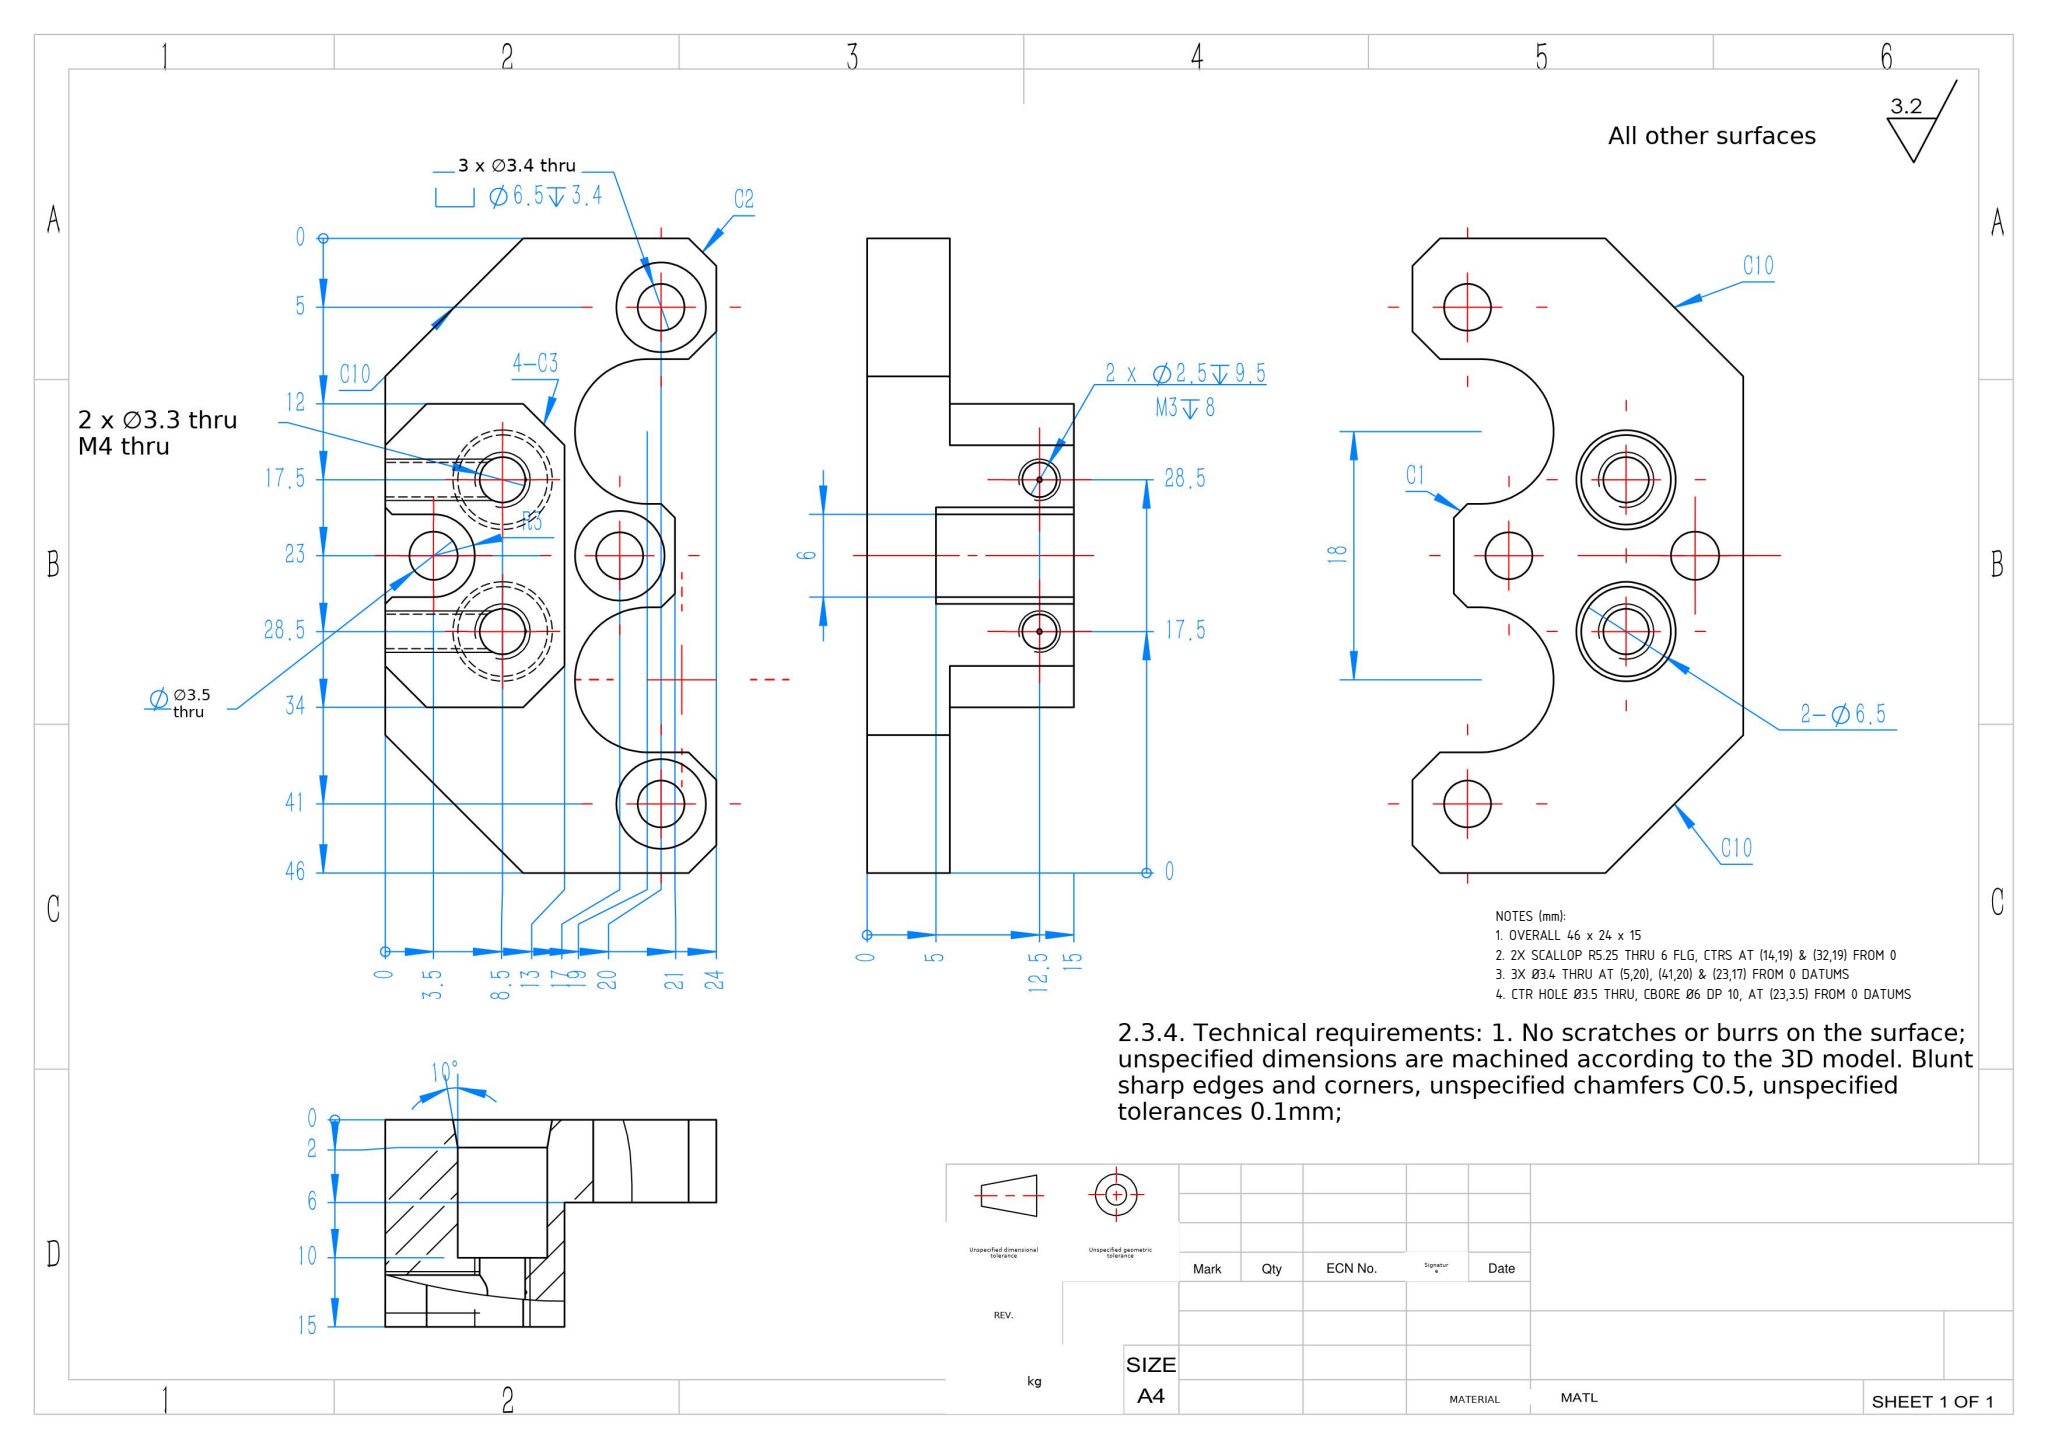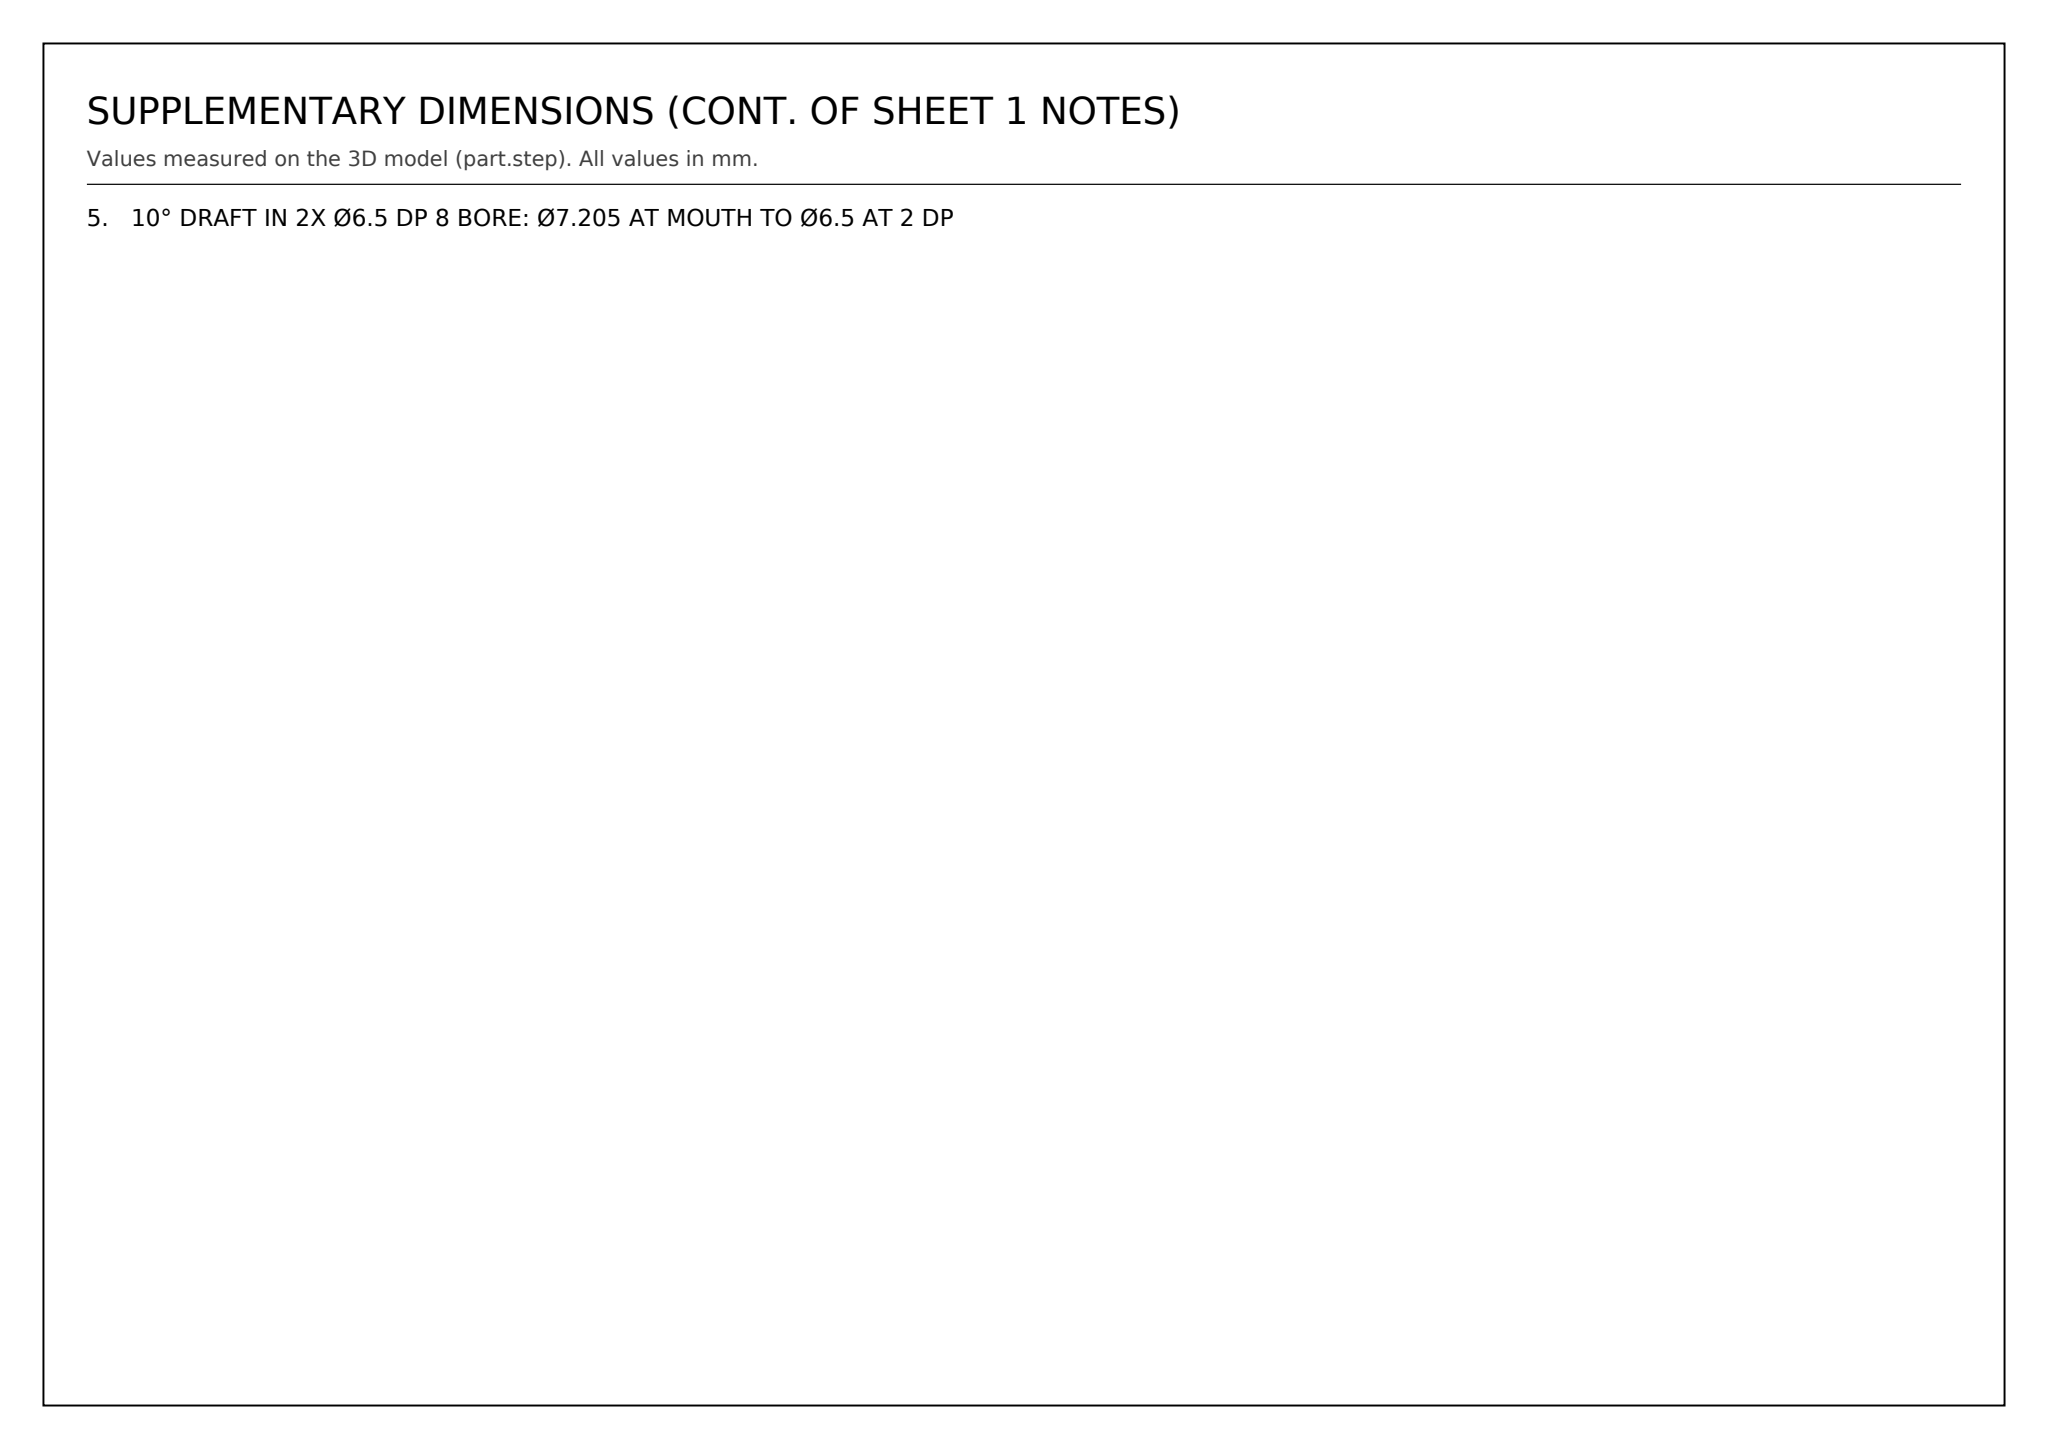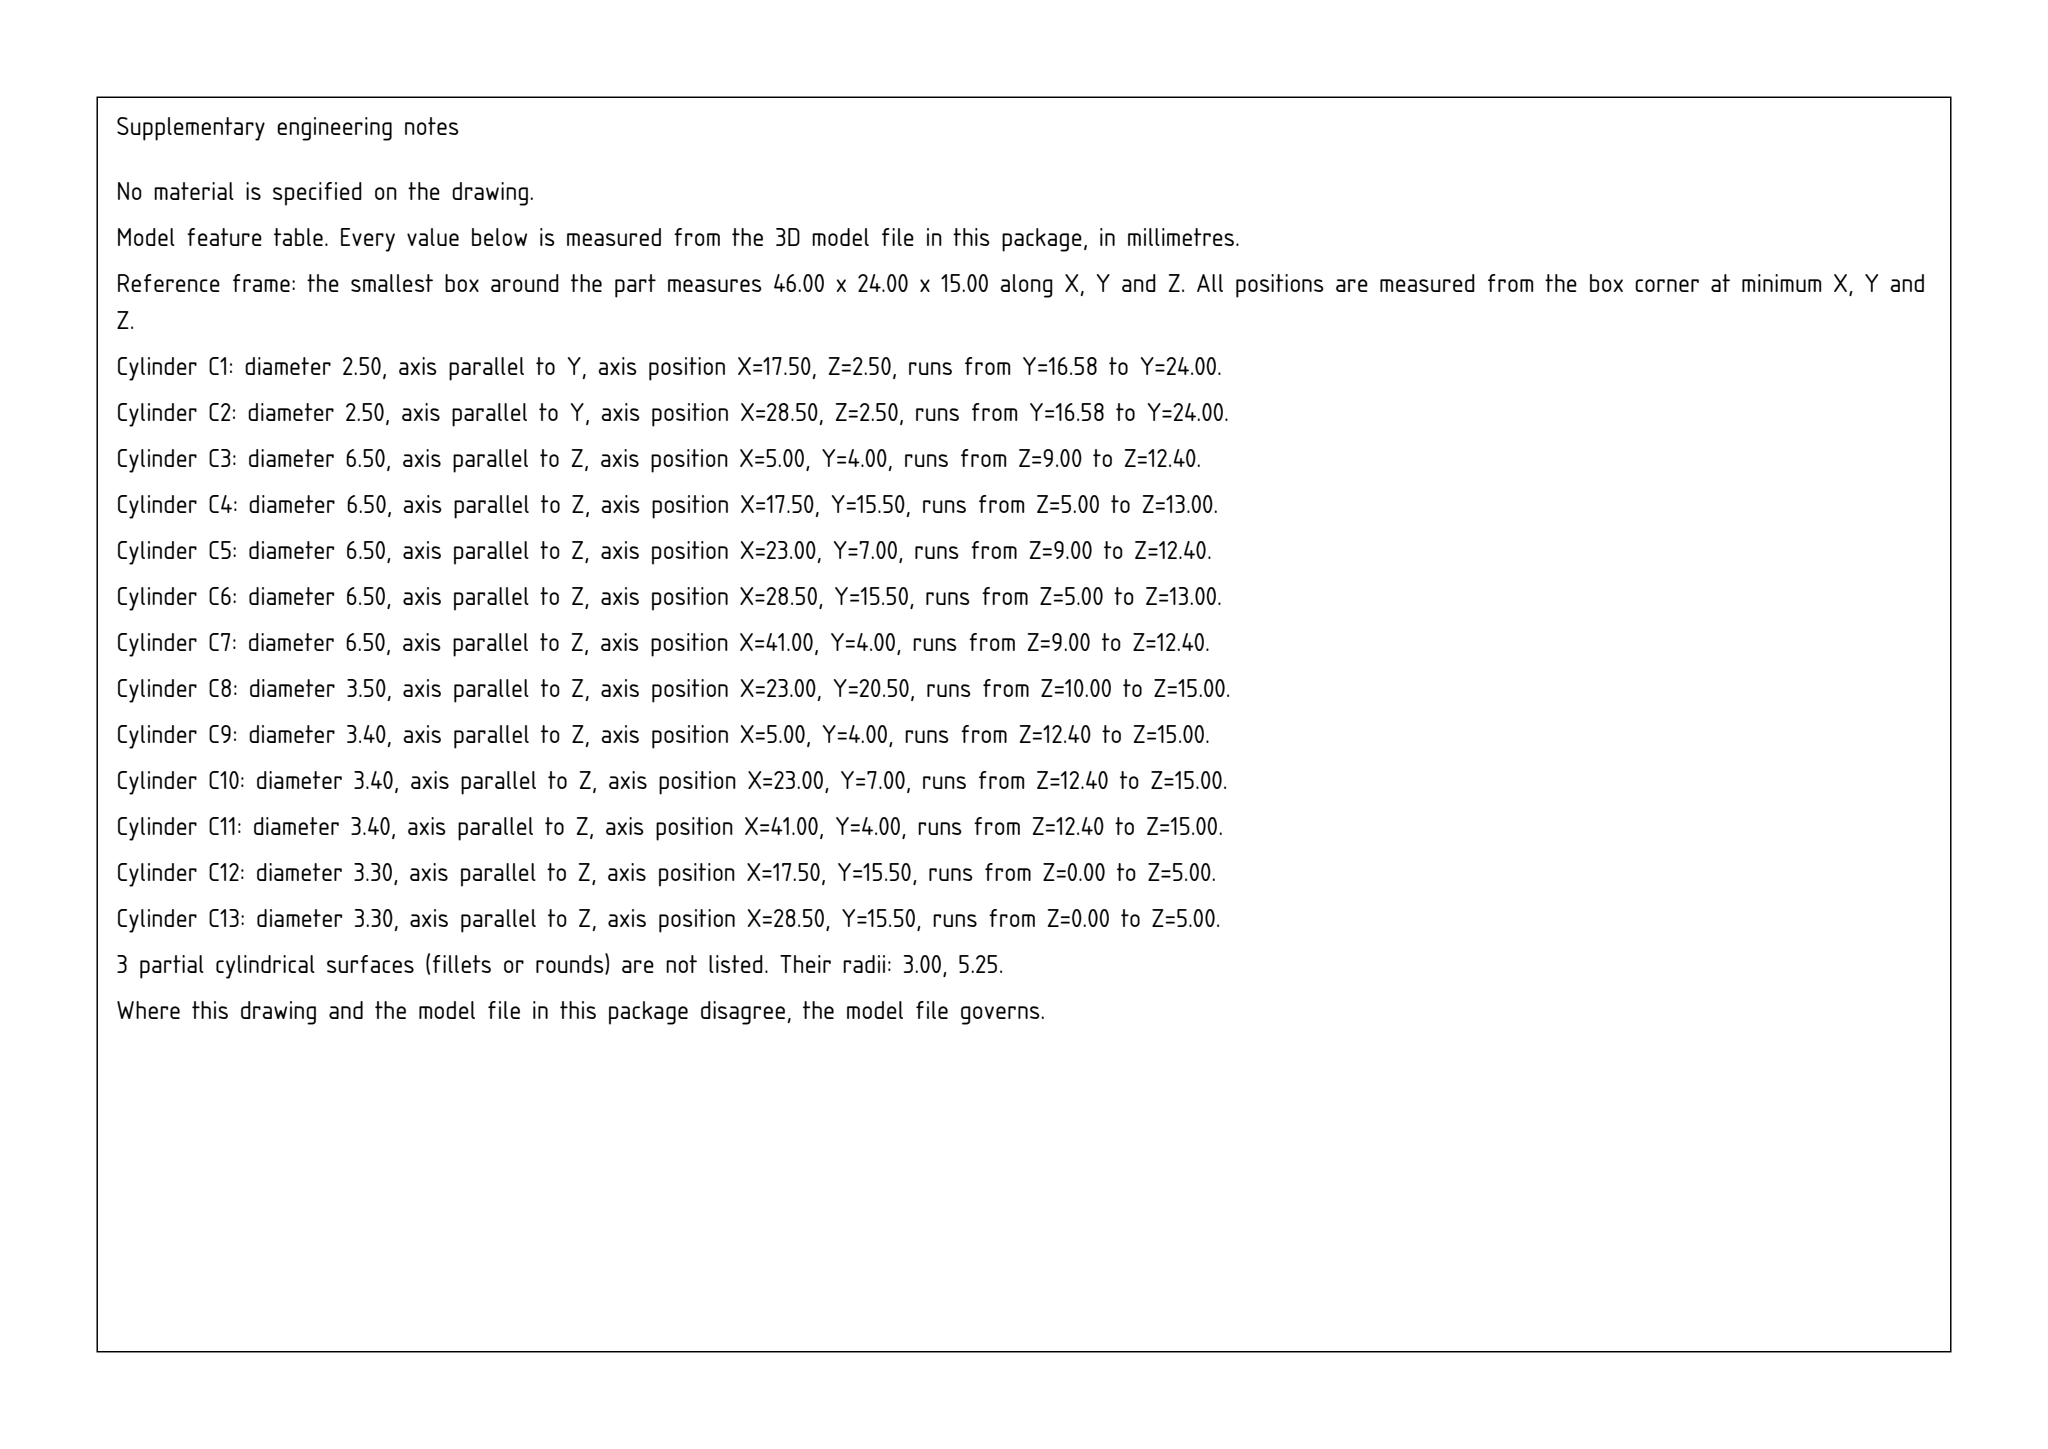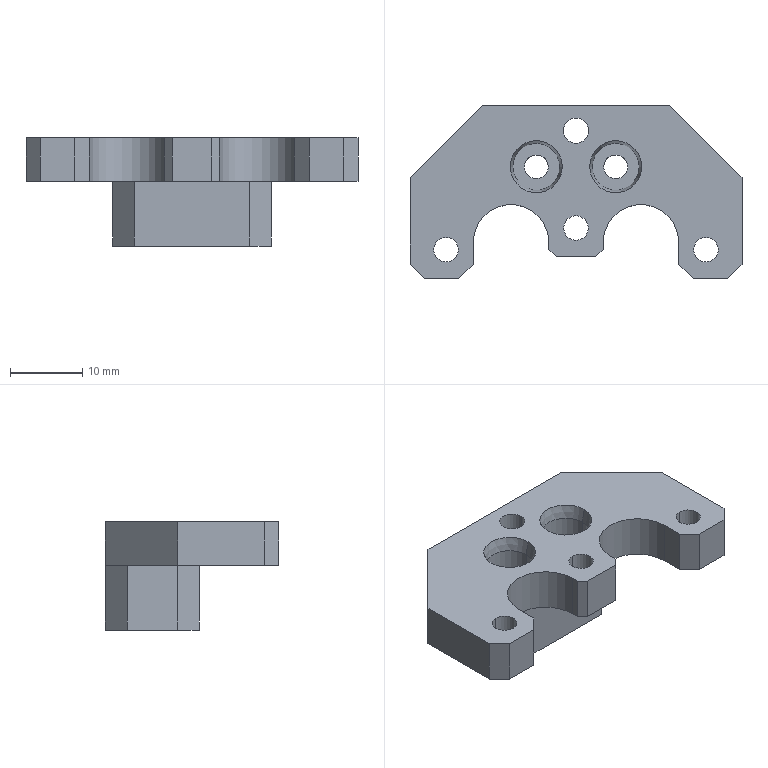Part | SolidWorks | mm | 1 solid | 75 faces | box 46 x 24 x 15 mm | volume 5454 mm3 | plane 38 | cylinder 29 | cone 8 | commonest cylinder face diameters 6.5 x10 3.4 x6 2.5 x4 3.3 x4 3.5 x2 10.5 x2 6 x1
Drawing notes:
OVERALL 46 x 24 x 15 | from the solid: bbox_xyz 46.0 x 24.0 x 15.0
2X SCALLOP R5.25 THRU 6 FLG, CTRS AT (14,19) & (32,19) FROM 0 | from the solid: cyl dia 10.5 axis z at (14,5) & (32,5), len 6 (flange z9-15); Y mirrored: 24-5=19
3X Ø3.4 THRU AT (5,20), (41,20) & (23,17) FROM 0 DATUMS | from the solid: cyl dia 3.4 axis z at (5,4),(41,4),(23,7) len 2.6 w/ Ø6.5 cbore; 24-4=20, 24-7=17
CTR HOLE Ø3.5 THRU, CBORE Ø6 DP 10, AT (23,3.5) FROM 0 DATUMS | from the solid: cyl dia 3.5 axis z at (23,20.5) len 5 + dia 6 same ctr len 10 = 15 thru; 24-20.5=3.5
10° DRAFT IN 2X Ø6.5 DP 8 BORE: Ø7.205 AT MOUTH TO Ø6.5 AT 2 DP | from the solid: cones incl 20.0, ref dia 7.205, qty 4 on Ø6.5 bores (17.5,15.5)&(28.5,15.5); (7.205-6.5)/2/tan10=2.0
build123d program:
from build123d import *
from OCP.BRepFilletAPI import BRepFilletAPI_MakeChamfer

# Parameters (mm, degrees)
SKETCH1_W                                       = 46
SKETCH1_H                                       = 24
BOSS_EXTRUDE1_DEPTH                             = 7.5
SKETCH10_W                                      = 9
SKETCH10_H                                      = 11
CUT_EXTRUDE3_DEPTH                              = 49.127
SKETCH2_R                                       = 3.25
CUT_EXTRUDE1_DEPTH                              = 10
M3_HEX_SOCKET_HEAD_CAP_SCREW_CBORE1_D           = 3.4
M3_HEX_SOCKET_HEAD_CAP_SCREW_CBORE1_CBORE_D     = 6.5
M3_HEX_SOCKET_HEAD_CAP_SCREW_CBORE1_CBORE_DEPTH = 3.4
CHAMFER1_SIZE                                   = 10
F_4_5_4_5_DIAMETER_HOLE1_D                      = 3.5
M4_TAPPED_HOLE1_D                               = 3.3
CHAMFER2_SIZE                                   = 2
CHAMFER2_SIZE2                                  = 0.3527
CUT_EXTRUDE2_DEPTH                              = 30.967
CHAMFER3_SIZE                                   = 2
CUT_EXTRUDE4_DEPTH                              = 10
CHAMFER4_SIZE                                   = 0.5
M3_TAPPED_HOLE2_D                               = 2.5
M3_TAPPED_HOLE2_DEPTH                           = 9.5
M3_TAPPED_HOLE2_TIP                             = 0.7511
SKETCH14_W                                      = 7.5
SKETCH14_H                                      = 3
CUT_EXTRUDE5_DEPTH                              = 28.459
CHAMFER5_SIZE                                   = 1
SKETCH15_W                                      = 12
SKETCH15_H                                      = 9
CUT_EXTRUDE6_DEPTH                              = 28.464
CHAMFER6_SIZE                                   = 3


with BuildPart() as part:
    # Sketch1 → Boss-Extrude1 (new, symmetric)
    with BuildSketch(Plane.XY):
        Rectangle(SKETCH1_W, SKETCH1_H)
    extrude(amount=BOSS_EXTRUDE1_DEPTH, both=True)

    # Sketch10 → Cut-Extrude3 (cut, through all)
    with BuildSketch(Plane(origin=(23, 0, 0), x_dir=(0, 0, -1), z_dir=(1, 0, 0))):
        with Locations((3, -6.5)):
            Rectangle(SKETCH10_W, SKETCH10_H)
    extrude(amount=-CUT_EXTRUDE3_DEPTH, mode=Mode.SUBTRACT)

    # Sketch2 → Cut-Extrude1 (cut)
    with BuildSketch(Plane(origin=(0, 0, 7.5), x_dir=(-1, 0, 0), z_dir=(0, 0, -1))):
        with Locations((-5.5, 3.5)):
            Circle(SKETCH2_R)
        with Locations((5.5, 3.5)):
            Circle(SKETCH2_R)
    extrude(amount=CUT_EXTRUDE1_DEPTH, mode=Mode.SUBTRACT)

    # M3 Hex Socket Head Cap Screw CBORE1 (through all)
    with Locations(Plane(origin=(0, 0, 1.5), x_dir=(-1, 0, 0), z_dir=(0, 0, -1))):
        with Locations((0, -5), (-18, -8), (18, -8)):
            CounterBoreHole(M3_HEX_SOCKET_HEAD_CAP_SCREW_CBORE1_D / 2, M3_HEX_SOCKET_HEAD_CAP_SCREW_CBORE1_CBORE_D / 2, M3_HEX_SOCKET_HEAD_CAP_SCREW_CBORE1_CBORE_DEPTH)

    # Chamfer1
    chamfer1_edges = [part.edges().sort_by_distance(p)[0] for p in [
        (-23, 12, 0),
        (23, 12, 0),
    ]]
    chamfer(chamfer1_edges, length=CHAMFER1_SIZE)

    # 4.5 _4.5_ Diameter Hole1 (through all)
    with Locations(Plane(origin=(0, 0, -7.5), x_dir=(-1, 0, 0), z_dir=(0, 0, -1))):
        with Locations((0, 8.5)):
            Hole(F_4_5_4_5_DIAMETER_HOLE1_D / 2)

    # M4 Tapped Hole1 (through all)
    with Locations(Plane.XY.offset(-2.5)):
        with Locations((5.5, 3.5), (-5.5, 3.5)):
            Hole(M4_TAPPED_HOLE1_D / 2)

    # Chamfer2: one chamfer whose edges measure the first distance from different faces: ONE call of the kernel's chamfer builder (chamfer() names one face for all edges)
    chamfer2_edges_1 = [part.edges().sort_by_distance(p)[0] for p in [
        (8.75, 3.5, 7.5),
    ]]
    chamfer2_side_1 = [part.faces().sort_by_distance(p)[0] for p in [
        (8.75, 3.5, 2.5),
    ]]
    chamfer2_edges_2 = [part.edges().sort_by_distance(p)[0] for p in [
        (-2.25, 3.5, 7.5),
    ]]
    chamfer2_side_2 = [part.faces().sort_by_distance(p)[0] for p in [
        (-2.25, 3.5, 2.5),
    ]]
    chamfer2 = BRepFilletAPI_MakeChamfer(part.part.solid().wrapped)
    for e in chamfer2_edges_1:
        chamfer2.Add(CHAMFER2_SIZE, CHAMFER2_SIZE2, e.wrapped, chamfer2_side_1[0].wrapped)  # the first distance lies on this face
    for e in chamfer2_edges_2:
        chamfer2.Add(CHAMFER2_SIZE, CHAMFER2_SIZE2, e.wrapped, chamfer2_side_2[0].wrapped)  # the first distance lies on this face
    add(Compound.cast(chamfer2.Shape()), mode=Mode.REPLACE)

    # Sketch9 → Cut-Extrude2 (cut, through all)
    with BuildSketch(Plane(origin=(0, 0, -7.5), x_dir=(-1, 0, 0), z_dir=(0, 0, -1))):
        with BuildLine():
            Line((-14.25, -12), (-14.25, -7))
            ThreePointArc((-14.25, -7), (-9, -1.75), (-3.75, -7))
            Line((-3.75, -7), (-3.75, -12))
            ThreePointArc((-3.75, -12), (-9, -17.25), (-14.25, -12))
        make_face()
        with BuildLine():
            Line((3.75, -12), (3.75, -7))
            ThreePointArc((3.75, -7), (9, -1.75), (14.25, -7))
            Line((14.25, -7), (14.25, -12))
            ThreePointArc((14.25, -12), (9, -17.25), (3.75, -12))
        make_face()
    extrude(amount=-CUT_EXTRUDE2_DEPTH, mode=Mode.SUBTRACT)

    # Chamfer3
    chamfer3_edges = [part.edges().sort_by_distance(p)[0] for p in [
        (14.25, -12, 4.5),
        (3.75, -12, 4.5),
        (-3.75, -12, 4.5),
        (-14.25, -12, 4.5),
        (23, -12, 4.5),
        (-23, -12, 4.5),
    ]]
    chamfer(chamfer3_edges, length=CHAMFER3_SIZE)

    # Sketch11 → Cut-Extrude4 (cut)
    with BuildSketch(Plane(origin=(0, 0, -7.5), x_dir=(-1, 0, 0), z_dir=(0, 0, -1))):
        with BuildLine():
            Line((-3, 8.5), (-3, 12))
            ThreePointArc((-3, 12), (0, 15), (3, 12))
            Line((3, 12), (3, 8.5))
            ThreePointArc((3, 8.5), (0, 5.5), (-3, 8.5))
        make_face()
    extrude(amount=-CUT_EXTRUDE4_DEPTH, mode=Mode.SUBTRACT)

    # Chamfer4
    chamfer4_edges = [part.edges().sort_by_distance(p)[0] for p in [
        (3, 12, -2.5),
        (-3, 12, -2.5),
    ]]
    chamfer(chamfer4_edges, length=CHAMFER4_SIZE)

    # M3 Tapped Hole2
    with Locations(Plane(origin=(0, 12, 0), x_dir=(1, 0, 0), z_dir=(0, 1, 0))):
        with Locations((5.5, 5), (-5.5, 5)):
            Hole(M3_TAPPED_HOLE2_D / 2, depth=M3_TAPPED_HOLE2_DEPTH)
            with Locations((0, 0, -(M3_TAPPED_HOLE2_DEPTH + M3_TAPPED_HOLE2_TIP / 2))):  # 118° drill point
                Cone(0, M3_TAPPED_HOLE2_D / 2, M3_TAPPED_HOLE2_TIP, mode=Mode.SUBTRACT)

    # Sketch14 → Cut-Extrude5 (cut, through all)
    with BuildSketch(Plane(origin=(0, 0, 1.5), x_dir=(-1, 0, 0), z_dir=(0, 0, -1))):
        with Locations((0, -10.5)):
            Rectangle(SKETCH14_W, SKETCH14_H)
    extrude(amount=-CUT_EXTRUDE5_DEPTH, mode=Mode.SUBTRACT)

    # Chamfer5
    chamfer5_edges = [part.edges().sort_by_distance(p)[0] for p in [
        (3.75, -9, 4.5),
        (-3.75, -9, 4.5),
    ]]
    chamfer(chamfer5_edges, length=CHAMFER5_SIZE)

    # Sketch15 → Cut-Extrude6 (cut, through all)
    with BuildSketch(Plane.XZ.offset(1)):
        with Locations((17, -3)):
            Rectangle(SKETCH15_W, SKETCH15_H)
        with Locations((-17, -3)):
            Rectangle(SKETCH15_W, SKETCH15_H)
    extrude(amount=-CUT_EXTRUDE6_DEPTH, mode=Mode.SUBTRACT)

    # Chamfer6
    chamfer6_edges = [part.edges().sort_by_distance(p)[0] for p in [
        (11, 12, -3),
        (11, -1, -3),
        (-11, 12, -3),
        (-11, -1, -3),
    ]]
    chamfer(chamfer6_edges, length=CHAMFER6_SIZE)


solid = part.part